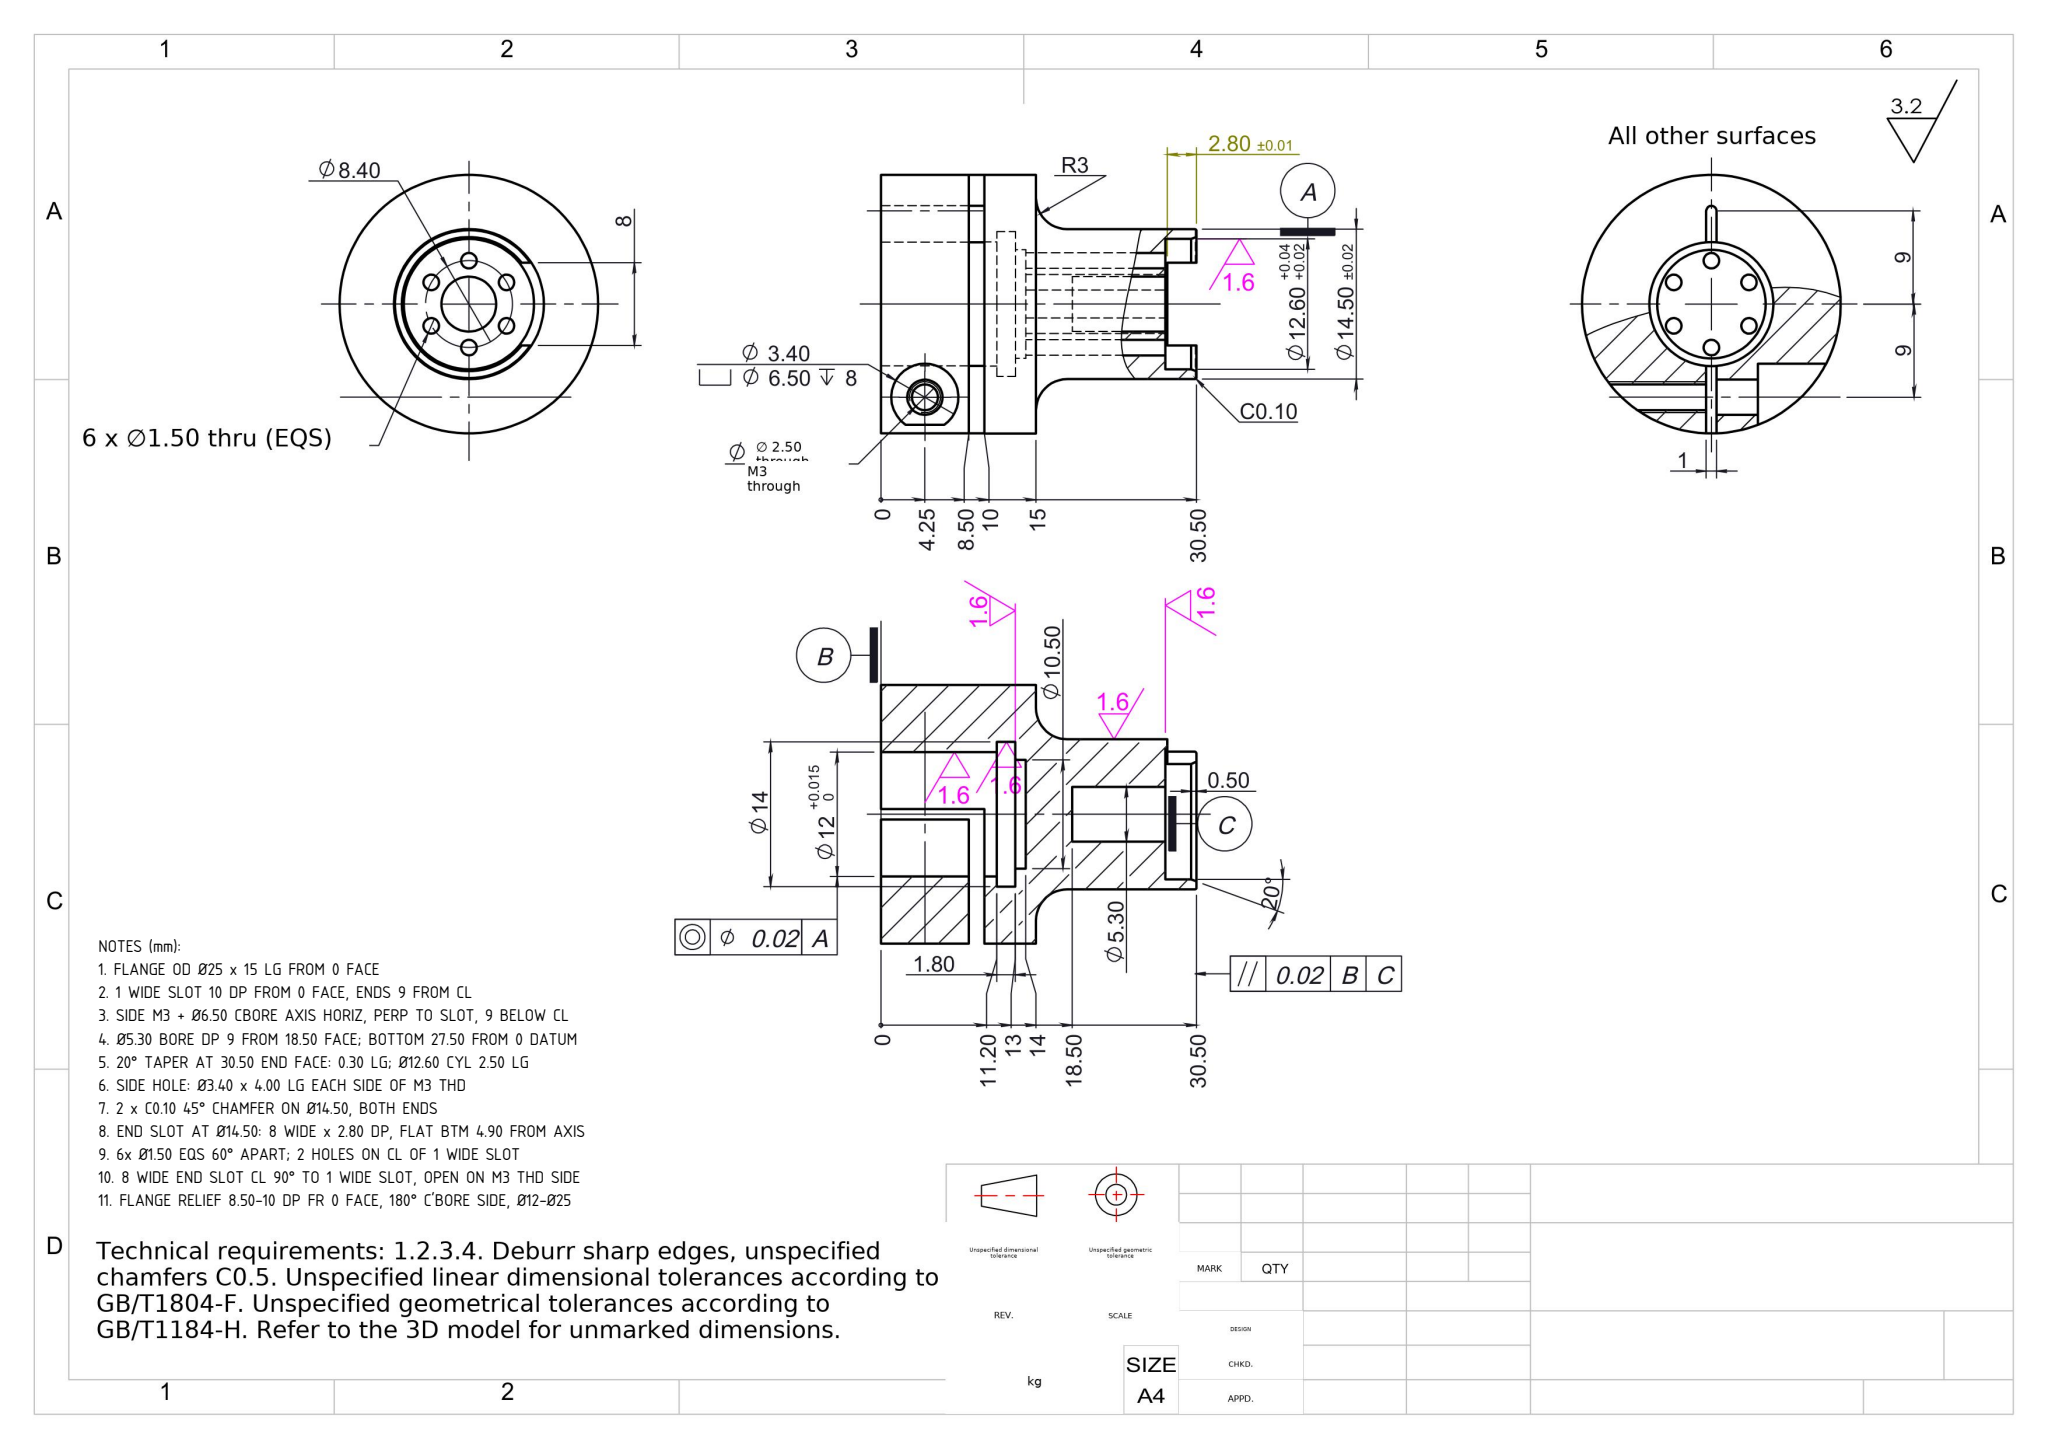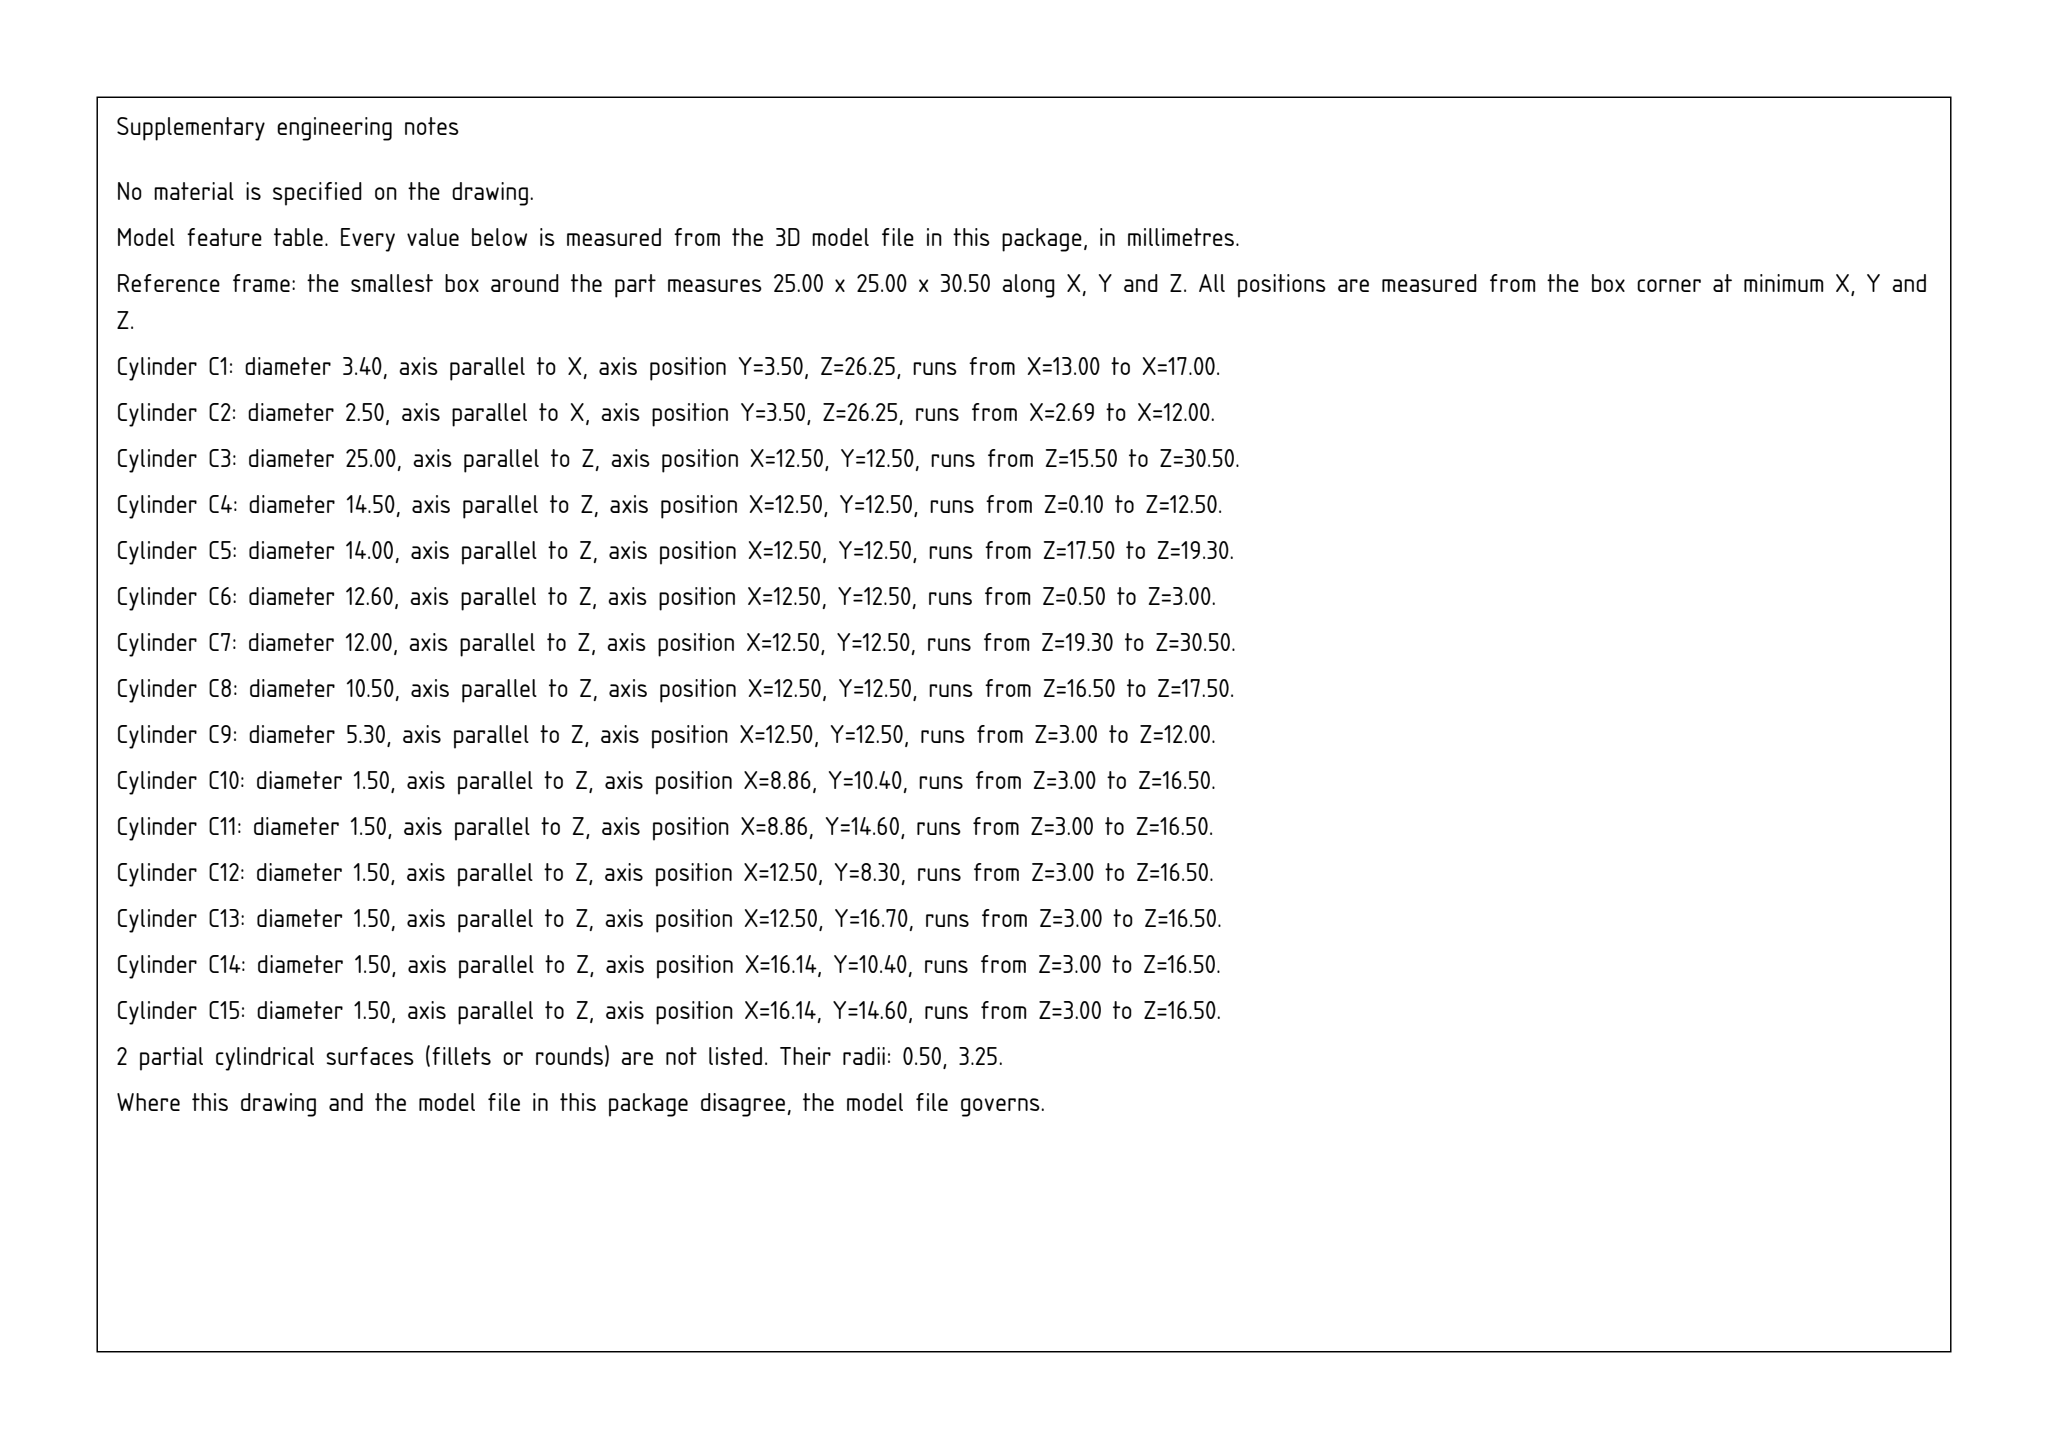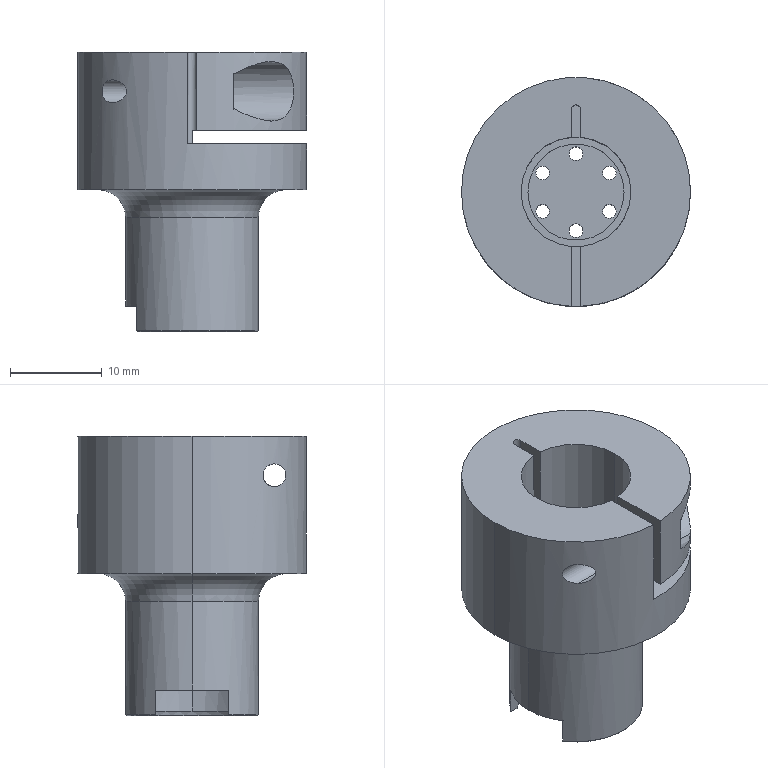Part | SolidWorks | mm | 1 solid | 61 faces | box 25 x 25 x 30.5 mm | volume 7070 mm3 | cylinder 37 | plane 19 | cone 3 | torus 2 | commonest cylinder face diameters 1.5 x12 12 x4 6.5 x3 25 x3 5.3 x2 12.6 x2 10.5 x2 2.5 x2
Drawing notes:
FLANGE OD Ø25 x 15 LG FROM 0 FACE | from the solid: cylinder dia 25.0, axis z, at (12.5,12.5), length 15 (z=15.5 to 30.5)
1 WIDE SLOT 10 DP FROM 0 FACE, ENDS 9 FROM CL | from the solid: Ø1 z-cyl at (12.5,21.5) L=10 (z=20.5 to 30.5), slot faces x=12.0/13.0; 21.5-12.5=9
SIDE M3 + Ø6.50 CBORE AXIS HORIZ, PERP TO SLOT, 9 BELOW CL | from the solid: x-axis cyls Ø2.5/Ø3.4/Ø6.5 at y=3.5, z=26.25; part axis y=12.5 -> 9 offset; slot normal x
Ø5.30 BORE DP 9 FROM 18.50 FACE; BOTTOM 27.50 FROM 0 DATUM | from the solid: cylinder [5.30, z, (12.5,12.5), length 9.0]; spans z=3.0-12.0, i.e. 18.50-27.50 from the 0 face (z=30.5)
20° TAPER AT 30.50 END FACE: 0.30 LG; Ø12.60 CYL 2.50 LG | from the solid: cone [40° incl = 20° half, ref dia 12.6] at z=0 end; Ø12.60 cyl length 2.5 within the 2.80 overall to plane z=2.8
SIDE HOLE: Ø3.40 x 4.00 LG EACH SIDE OF M3 THD | from the solid: cylinders [3.4, x, (y3.5,z26.25), length 4.0, count 2] flanking Ø2.50/M3 through
2 x C0.10 45° CHAMFER ON Ø14.50, BOTH ENDS | from the solid: cones [90.0 incl, ref dia 14.5, count 2] at both ends of Ø14.50 x 12.4 cyl
END SLOT AT Ø14.50: 8 WIDE x 2.80 DP, FLAT BTM 4.90 FROM AXIS | from the solid: y-planes at y=8.5 and y=16.5 (8 apart, straddling axis y=12.5), x[6.5,7.6], z[0,2.8]; slot floor plane z=2.8 (x 5.3-7.6, y 8.5-16.5); bottom flat at x=7.6 = 4.90 from axis x=12.5 (2.35 deep into Ø14.50)
6x Ø1.50 EQS 60° APART; 2 HOLES ON CL OF 1 WIDE SLOT | from the solid: Ø1.5 holes at (12.5,16.7),(12.5,8.3),(16.1,14.6),(16.1,10.4),(8.9,14.6),(8.9,10.4) about axis (12.5,12.5) = 30/90/150/210/270/330° on Ø8.4 BC; 1 wide slot bounded by x=12.0 and x=13.0 planes, CL x=12.5 along y, R0.5 end at (12.5,21.5)
8 WIDE END SLOT CL 90° TO 1 WIDE SLOT, OPEN ON M3 THD SIDE | from the solid: End slot walls y=8.5 & y=16.5 (8 wide, symm about axis y=12.5), floor z=2.8, inner wall x=7.6 (4.9 from axis), open toward -X at OD; 1 wide slit lies x=12.0-13.0 (plane normal X); M3 Ø2.5 thd x=2.7-12.0 on -X side, Ø6.5 c'bore x=17.0-23.6 on +X side -> slot length dir parallel to M3 axis, 90° to slit plane, opening on thread side
FLANGE RELIEF 8.50-10 DP FR 0 FACE, 180° C'BORE SIDE, Ø12-Ø25 | from the solid: Flange 0-face = model z=30.5; faces z=20.5 (area 194, bbox x[12,25]) and z=22.0 (area 184, bbox x[12.5,25]) = half-annulus Ø12 to Ø25 on +X (c'bore) half; 30.5-20.5=10 dp slot floor, 30.5-22.0=8.50 dp second floor, 1.50 step
build123d program:
from build123d import *

# Parameters (mm, degrees)
SKETCH1_R                                       = 7.25
BOSS_EXTRUDE1_DEPTH                             = 18
SKETCH6_W                                       = 37.803
SKETCH6_H                                       = 15
CUT_EXTRUDE1_DEPTH                              = 2.5
SKETCH11_R                                      = 12.5
BOSS_EXTRUDE2_DEPTH                             = 15
SKETCH12_W                                      = 17.519
SKETCH12_H                                      = 1.5
CUT_EXTRUDE4_DEPTH                              = 22.5
CUT_EXTRUDE5_REACH                              = 37.253
SKETCH14_R                                      = 6
CUT_EXTRUDE6_DEPTH                              = 14
CUT_EXTRUDE7_START                              = 1
SKETCH15_R                                      = 7
CUT_EXTRUDE7_DEPTH                              = 1.8
M3_HEX_SOCKET_HEAD_CAP_SCREW_CBORE1_D           = 3.4
M3_HEX_SOCKET_HEAD_CAP_SCREW_CBORE1_DEPTH       = 12
M3_HEX_SOCKET_HEAD_CAP_SCREW_CBORE1_CBORE_D     = 6.5
M3_HEX_SOCKET_HEAD_CAP_SCREW_CBORE1_CBORE_DEPTH = 8
M3_TAPPED_HOLE1_D                               = 2.5
BOSS_EXTRUDE3_START                             = 1
SKETCH20_R                                      = 6
SKETCH20_R_2                                    = 5.25
BOSS_EXTRUDE3_DEPTH                             = 1
FILLET2_R                                       = 3
SKETCH10_R                                      = 2.65
CUT_EXTRUDE8_DEPTH                              = 12
SKETCH21_R                                      = 6.3
CUT_EXTRUDE9_DEPTH                              = 3
SIZE_MM_DOWEL_PIN_HOLE_0_D                      = 1.5
CIRPATTERN1_COUNT                               = 6
CHAMFER1_SIZE                                   = 0.5
CHAMFER1_SIZE2                                  = 0.182
SKETCH24_W                                      = 5.178
SKETCH24_H                                      = 8
CUT_EXTRUDE10_DEPTH                             = 2.8
CHAMFER2_SIZE                                   = 0.1


with BuildPart() as part:
    # Sketch1 → Boss-Extrude1 (new body)
    with BuildSketch(Plane.XY):
        Circle(SKETCH1_R)
    extrude(amount=BOSS_EXTRUDE1_DEPTH)

    # Sketch6 → Cut-Extrude1 (cut)
    with BuildSketch(Plane(origin=(0, 0, 0), x_dir=(-1, 0, 0), z_dir=(0, 0, -1))):
        Rectangle(SKETCH6_W, SKETCH6_H)
    extrude(amount=-CUT_EXTRUDE1_DEPTH, mode=Mode.SUBTRACT)

    # Sketch11 → Boss-Extrude2 (add)
    with BuildSketch(Plane.XY.offset(18)):
        Circle(SKETCH11_R)
    extrude(amount=BOSS_EXTRUDE2_DEPTH)

    # Sketch12 → Cut-Extrude4 (cut, symmetric)
    with BuildSketch(Plane(origin=(0, 0, 0), x_dir=(1, 0, 0), z_dir=(0, 1, 0))):
        with Locations((8.76, -23.75)):
            Rectangle(SKETCH12_W, SKETCH12_H)
    extrude(amount=CUT_EXTRUDE4_DEPTH, both=True, mode=Mode.SUBTRACT)

    # Cut-Extrude5: up to this face of the body (flat: up to its plane)
    cut_extrude5_end = Plane(part.part.faces().sort_by_distance((5.305, 0, 23))[0])
    # Sketch13 → Cut-Extrude5 (cut, up to the picked face)
    with BuildSketch(Plane.XY.offset(33), mode=Mode.PRIVATE) as cut_extrude5_sk1:
        with BuildLine():
            Line((-0.5, -17.447), (-0.5, 9))
            ThreePointArc((-0.5, 9), (0, 9.5), (0.5, 9))
            Line((0.5, 9), (0.5, -17.447))
            ThreePointArc((0.5, -17.447), (0, -17.947), (-0.5, -17.447))
        make_face()
    cut_extrude5_tool1 = split(extrude(cut_extrude5_sk1.sketch, amount=-CUT_EXTRUDE5_REACH, mode=Mode.PRIVATE), bisect_by=cut_extrude5_end, keep=Keep.BOTH, mode=Mode.PRIVATE)
    add(cut_extrude5_tool1.solids().sort_by(Axis((0, -4.224, 33), (0, 0, -1)))[0], mode=Mode.SUBTRACT)

    # Sketch14 → Cut-Extrude6 (cut)
    with BuildSketch(Plane.XY.offset(33)):
        Circle(SKETCH14_R)
    extrude(amount=-CUT_EXTRUDE6_DEPTH, mode=Mode.SUBTRACT)

    # Sketch15 → Cut-Extrude7 (cut)
    with BuildSketch(Plane.XY.offset(19).offset(CUT_EXTRUDE7_START)):
        Circle(SKETCH15_R)
    extrude(amount=CUT_EXTRUDE7_DEPTH, mode=Mode.SUBTRACT)

    # M3 Hex Socket Head Cap Screw CBORE1
    with Locations(Plane(origin=(12.5, 0, 0), x_dir=(0, 0, -1), z_dir=(1, 0, 0))):
        with Locations((-28.75, -9)):
            CounterBoreHole(M3_HEX_SOCKET_HEAD_CAP_SCREW_CBORE1_D / 2, M3_HEX_SOCKET_HEAD_CAP_SCREW_CBORE1_CBORE_D / 2, M3_HEX_SOCKET_HEAD_CAP_SCREW_CBORE1_CBORE_DEPTH, depth=M3_HEX_SOCKET_HEAD_CAP_SCREW_CBORE1_DEPTH)

    # M3 Tapped Hole1 (through all)
    with Locations(Plane(origin=(-0.5, 0, 0), x_dir=(0, 0, -1), z_dir=(1, 0, 0))):
        with Locations((-28.75, -9)):
            Hole(M3_TAPPED_HOLE1_D / 2)

    # Sketch20 → Boss-Extrude3 (add)
    with BuildSketch(Plane.XY.offset(19).offset(BOSS_EXTRUDE3_START)):
        Circle(SKETCH20_R)
        Circle(SKETCH20_R_2, mode=Mode.SUBTRACT)
    extrude(amount=-BOSS_EXTRUDE3_DEPTH)

    # Fillet2
    fillet2_edges = [part.edges().sort_by_distance(p)[0] for p in [
        (-7.25, 0, 18),
    ]]
    fillet(fillet2_edges, radius=FILLET2_R)

    # Sketch10 → Cut-Extrude8 (cut)
    with BuildSketch(Plane(origin=(0, 0, 2.5), x_dir=(-1, 0, 0), z_dir=(0, 0, -1))):
        Circle(SKETCH10_R)
    extrude(amount=-CUT_EXTRUDE8_DEPTH, mode=Mode.SUBTRACT)

    # Sketch21 → Cut-Extrude9 (cut)
    with BuildSketch(Plane(origin=(0, 0, 2.5), x_dir=(-1, 0, 0), z_dir=(0, 0, -1))):
        Circle(SKETCH21_R)
    extrude(amount=-CUT_EXTRUDE9_DEPTH, mode=Mode.SUBTRACT)

    # Size mm Dowel Pin Hole 0 (through all)
    with Locations(Plane(origin=(0, 0, 5.5), x_dir=(-1, 0, 0), z_dir=(0, 0, -1))):
        with Locations((0, -4.2)):
            size_mm_dowel_pin_hole_0 = Hole(SIZE_MM_DOWEL_PIN_HOLE_0_D / 2)

    # CirPattern1: Size mm Dowel Pin Hole 0 ×6 about axis
    cirpattern1_axis = Axis((0, 0, 0), (0, 0, 1))
    for i in range(1, CIRPATTERN1_COUNT):
        add(size_mm_dowel_pin_hole_0.rotate(cirpattern1_axis, i * 360 / CIRPATTERN1_COUNT), mode=Mode.SUBTRACT)

    # Chamfer1
    chamfer1_edges = [part.edges().sort_by_distance(p)[0] for p in [
        (6.3, 0, 2.5),
    ]]
    chamfer1_side = [part.faces().sort_by_distance(p)[0] for p in [
        (6.3, 0, 4),
    ]]
    chamfer(chamfer1_edges, length=CHAMFER1_SIZE, length2=CHAMFER1_SIZE2, reference=chamfer1_side[0])

    # Sketch24 → Cut-Extrude10 (cut)
    with BuildSketch(Plane(origin=(0, 0, 2.5), x_dir=(-1, 0, 0), z_dir=(0, 0, -1))):
        with Locations((6.634, 0)):
            Rectangle(SKETCH24_W, SKETCH24_H)
    extrude(amount=-CUT_EXTRUDE10_DEPTH, mode=Mode.SUBTRACT)

    # Chamfer2
    chamfer2_edges = [part.edges().sort_by_distance(p)[0] for p in [
        (2.089, -6.943, 2.5),
    ]]
    chamfer(chamfer2_edges, length=CHAMFER2_SIZE)


solid = part.part